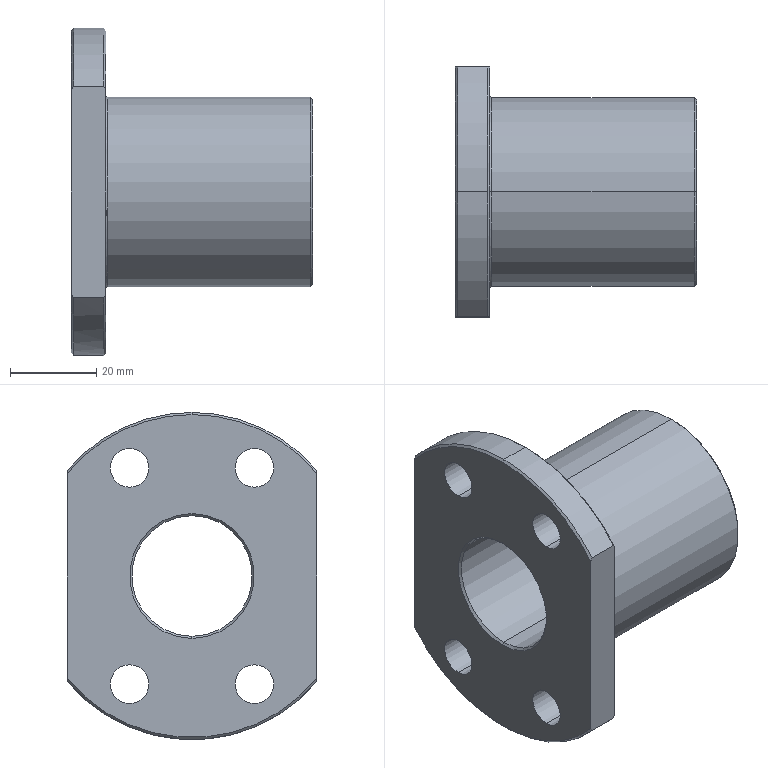Component | SolidWorks | TC020.05-05-1 | 1 solid | 34 faces | volume 67852 mm3 | cylinder 15 | cone 12 | plane 5 | spline 2 | commonest cylinder face diameters 9 x8 76 x3 28 x2 44 x2 | material H68